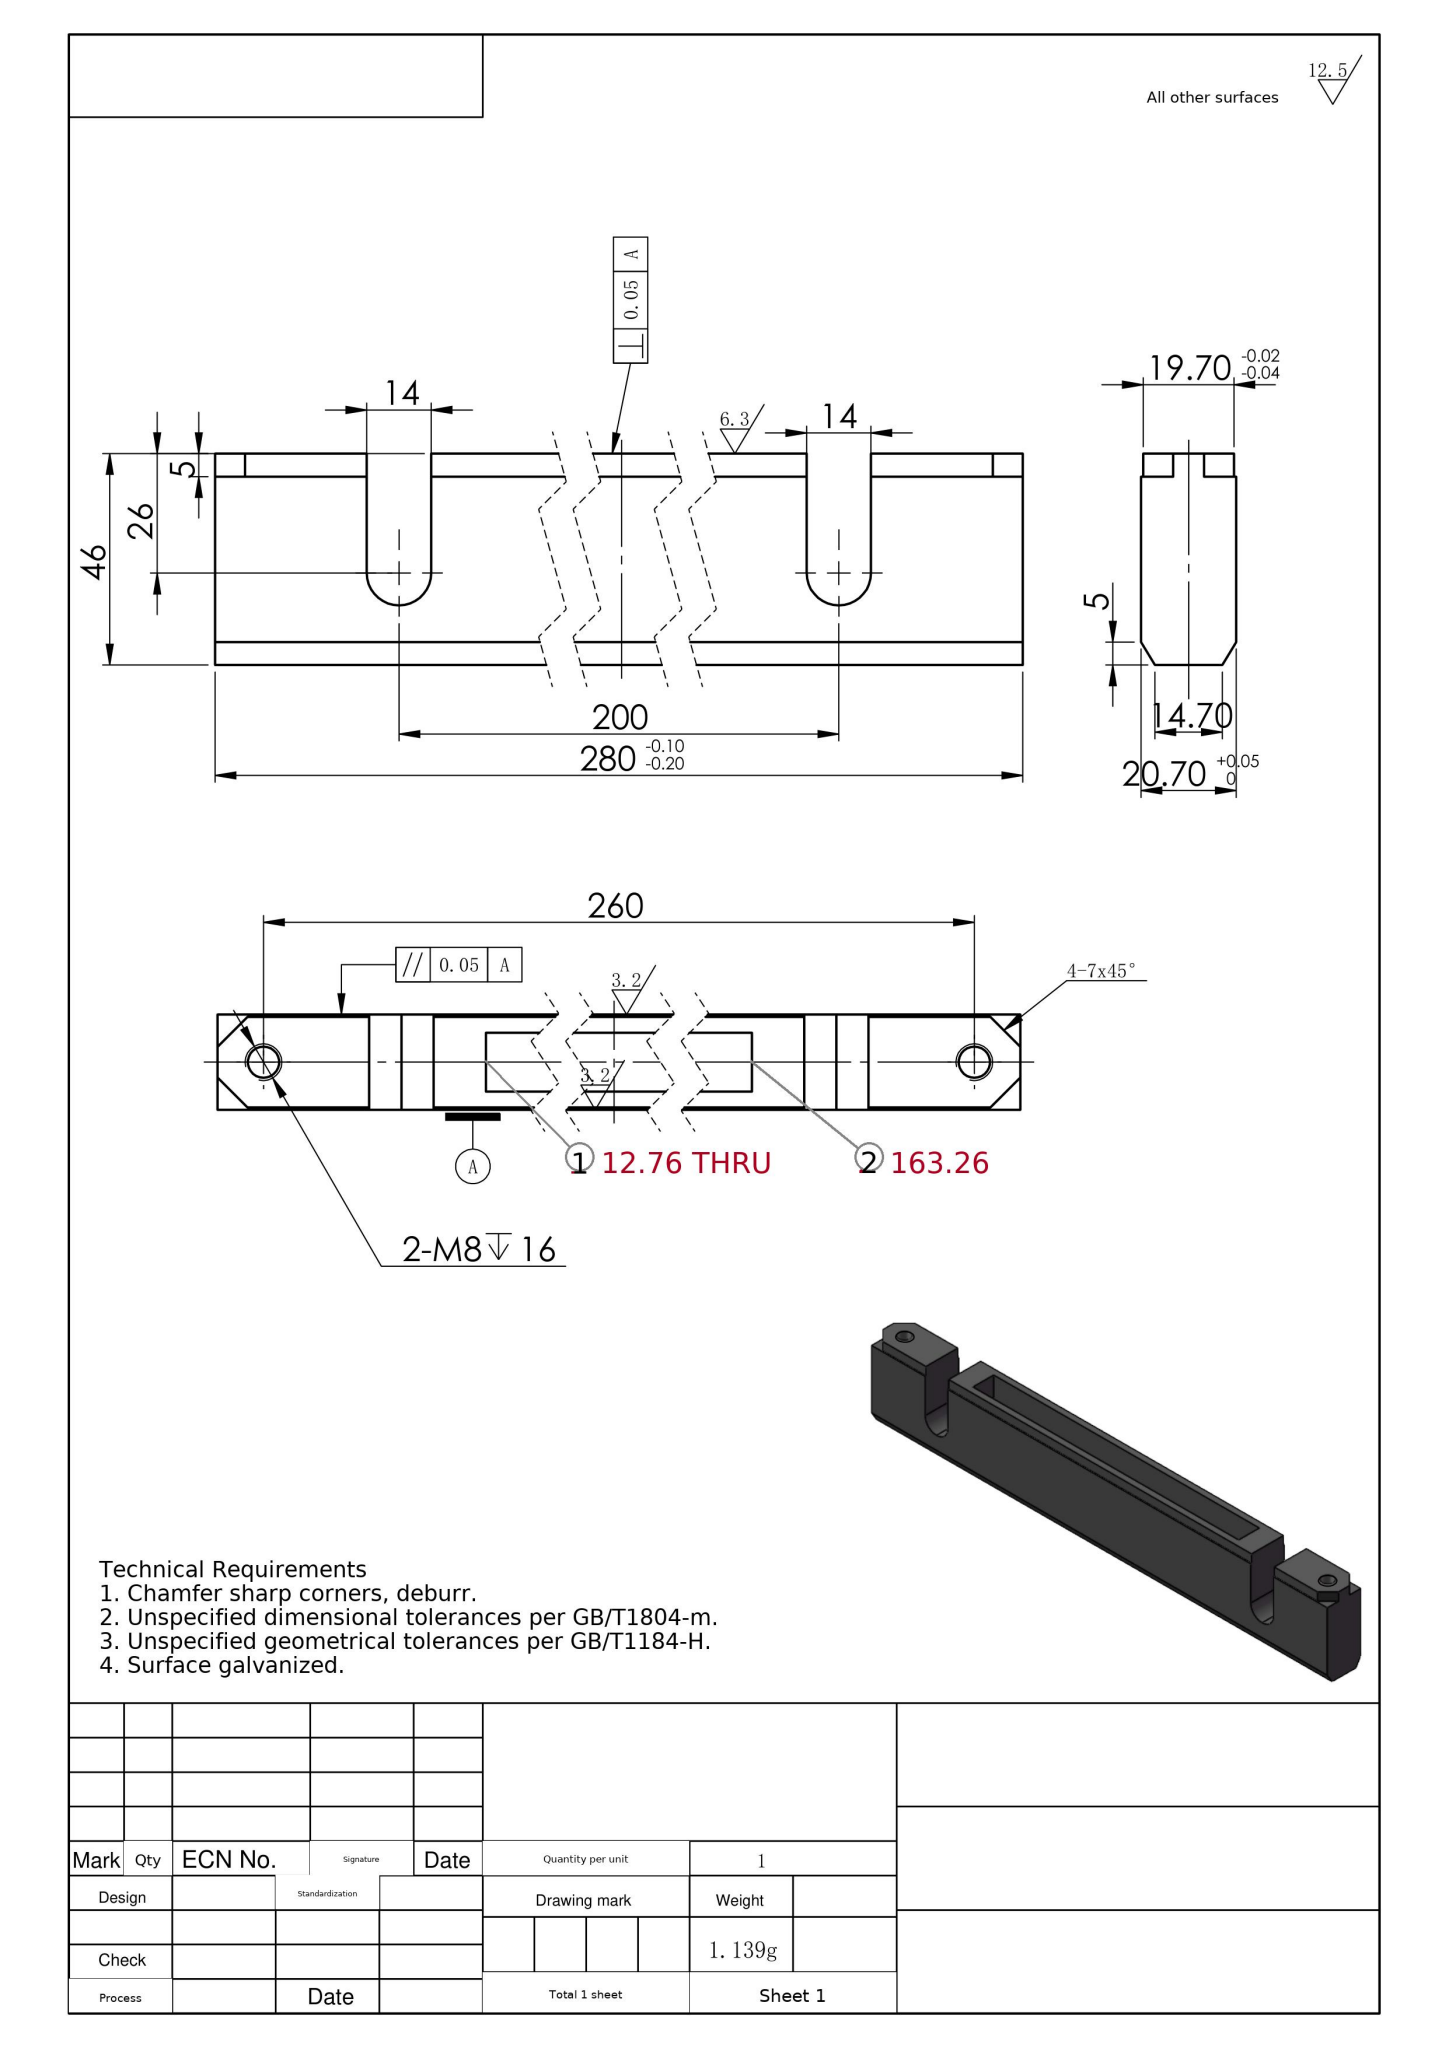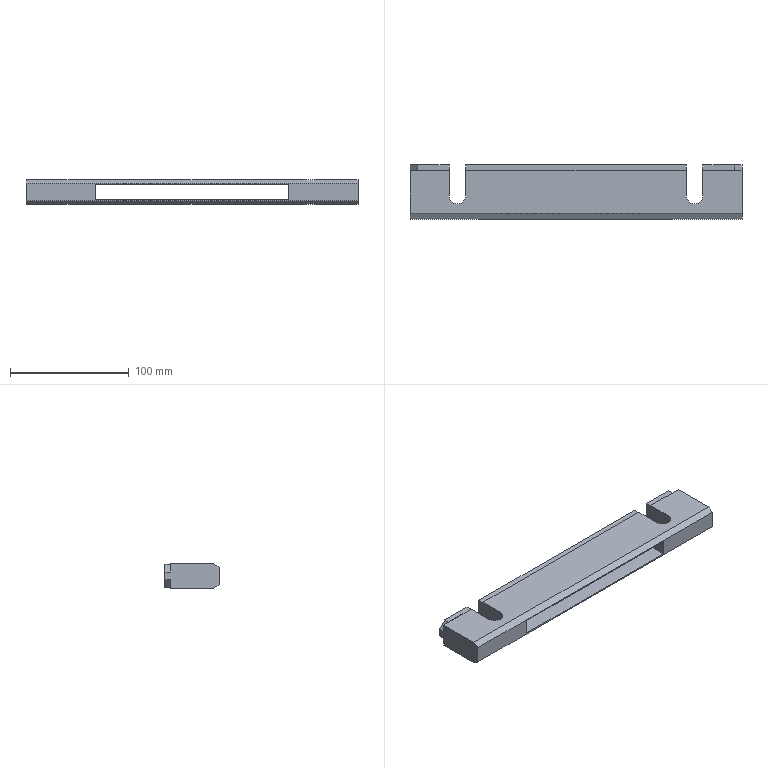Part | SolidWorks | mm | 1 solid | 46 faces | box 280 x 46 x 20.7 mm | volume 145134 mm3 | plane 34 | cylinder 8 | cone 4 | commonest cylinder face diameters 6.8 x4 14 x4